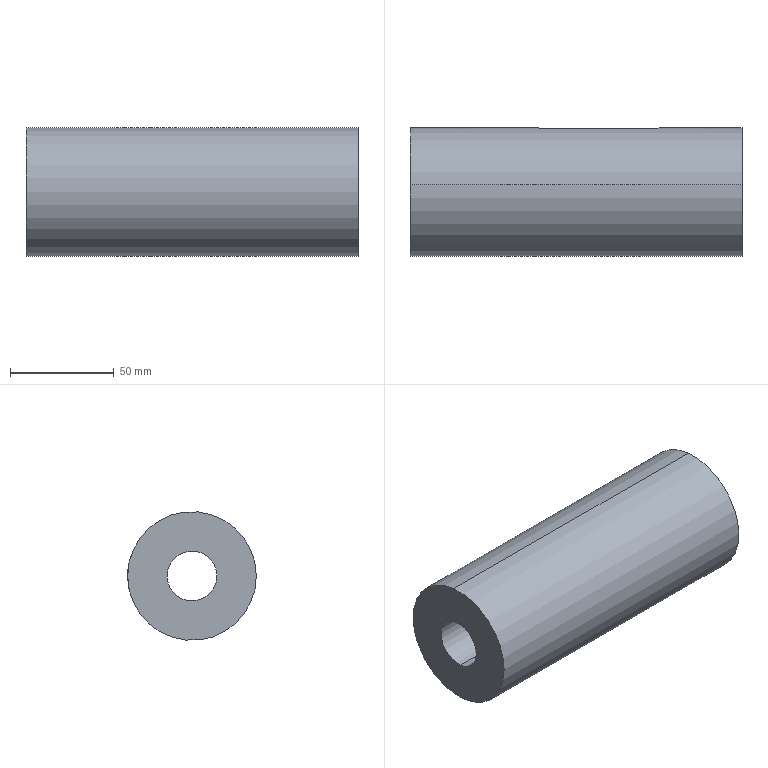Component | SolidWorks | Part4^LatheTailstock-1 | 1 solid | 17 faces | box 160 x 62 x 62 mm | volume 398970 mm3 | plane 9 | cylinder 8 | commonest cylinder face diameters 24 x4 30 x2 62 x2
STEP:
#1=CARTESIAN_POINT('',(-0.4506,5.972,-0.003713));
#2=VERTEX_POINT('',#1);
#3=CARTESIAN_POINT('',(-0.4506,5.839,-1.177));
#4=VERTEX_POINT('',#3);
#5=CARTESIAN_POINT('',(-0.4506,5.906,-0.5906));
#6=DIRECTION('',(1.,0.,0.));
#7=DIRECTION('',(0.,-0.112,-0.9937));
#8=AXIS2_PLACEMENT_3D('',#5,#6,#7);
#9=CIRCLE('',#8,0.5906);
#10=EDGE_CURVE('',#2,#4,#9,.T.);
#11=ORIENTED_EDGE('',*,*,#10,.F.);
#12=CARTESIAN_POINT('',(0.7305,5.972,-0.003713));
#13=VERTEX_POINT('',#12);
#14=CARTESIAN_POINT('',(-0.4506,5.972,-0.003713));
#15=DIRECTION('',(1.,0.,0.));
#16=VECTOR('',#15,39.37);
#17=LINE('',#14,#16);
#18=EDGE_CURVE('',#2,#13,#17,.T.);
#19=ORIENTED_EDGE('',*,*,#18,.T.);
#20=CARTESIAN_POINT('',(0.7305,5.839,-1.177));
#21=VERTEX_POINT('',#20);
#22=CARTESIAN_POINT('',(0.7305,5.906,-0.5906));
#23=DIRECTION('',(1.,0.,0.));
#24=DIRECTION('',(0.,-0.112,-0.9937));
#25=AXIS2_PLACEMENT_3D('',#22,#23,#24);
#26=CIRCLE('',#25,0.5906);
#27=EDGE_CURVE('',#13,#21,#26,.T.);
#28=ORIENTED_EDGE('',*,*,#27,.T.);
#29=CARTESIAN_POINT('',(-0.4506,5.839,-1.177));
#30=DIRECTION('',(1.,0.,0.));
#31=VECTOR('',#30,39.37);
#32=LINE('',#29,#31);
#33=EDGE_CURVE('',#4,#21,#32,.T.);
#34=ORIENTED_EDGE('',*,*,#33,.F.);
#35=EDGE_LOOP('',(#11,#19,#28,#34));
#36=FACE_OUTER_BOUND('',#35,.T.);
#37=CARTESIAN_POINT('',(-0.4506,5.906,-0.5906));
#38=DIRECTION('',(1.,0.,0.));
#39=DIRECTION('',(0.,-0.112,-0.9937));
#40=AXIS2_PLACEMENT_3D('',#37,#38,#39);
#41=CYLINDRICAL_SURFACE('',#40,0.5906);
#42=ADVANCED_FACE('',(#36),#41,.F.);
#43=CARTESIAN_POINT('',(0.7305,5.853,-1.06));
#44=VERTEX_POINT('',#43);
#45=CARTESIAN_POINT('',(0.7305,5.958,-0.1211));
#46=VERTEX_POINT('',#45);
#47=CARTESIAN_POINT('',(0.7305,5.906,-0.5906));
#48=DIRECTION('',(-1.,0.,0.));
#49=DIRECTION('',(0.,-0.112,-0.9937));
#50=AXIS2_PLACEMENT_3D('',#47,#48,#49);
#51=CIRCLE('',#50,0.4724);
#52=EDGE_CURVE('',#44,#46,#51,.T.);
#53=ORIENTED_EDGE('',*,*,#52,.T.);
#54=CARTESIAN_POINT('',(2.305,5.958,-0.1211));
#55=VERTEX_POINT('',#54);
#56=CARTESIAN_POINT('',(-3.207,5.958,-0.1211));
#57=DIRECTION('',(1.,0.,0.));
#58=VECTOR('',#57,39.37);
#59=LINE('',#56,#58);
#60=EDGE_CURVE('',#46,#55,#59,.T.);
#61=ORIENTED_EDGE('',*,*,#60,.T.);
#62=CARTESIAN_POINT('',(2.305,5.853,-1.06));
#63=VERTEX_POINT('',#62);
#64=CARTESIAN_POINT('',(2.305,5.906,-0.5906));
#65=DIRECTION('',(1.,0.,0.));
#66=DIRECTION('',(0.,-0.112,-0.9937));
#67=AXIS2_PLACEMENT_3D('',#64,#65,#66);
#68=CIRCLE('',#67,0.4724);
#69=EDGE_CURVE('',#55,#63,#68,.T.);
#70=ORIENTED_EDGE('',*,*,#69,.T.);
#71=CARTESIAN_POINT('',(-3.207,5.853,-1.06));
#72=DIRECTION('',(1.,0.,0.));
#73=VECTOR('',#72,39.37);
#74=LINE('',#71,#73);
#75=EDGE_CURVE('',#44,#63,#74,.T.);
#76=ORIENTED_EDGE('',*,*,#75,.F.);
#77=EDGE_LOOP('',(#53,#61,#70,#76));
#78=FACE_OUTER_BOUND('',#77,.T.);
#79=CARTESIAN_POINT('',(-3.207,5.906,-0.5906));
#80=DIRECTION('',(1.,0.,0.));
#81=DIRECTION('',(0.,-0.112,-0.9937));
#82=AXIS2_PLACEMENT_3D('',#79,#80,#81);
#83=CYLINDRICAL_SURFACE('',#82,0.4724);
#84=ADVANCED_FACE('',(#78),#83,.F.);
#85=CARTESIAN_POINT('',(-3.994,5.853,-1.06));
#86=VERTEX_POINT('',#85);
#87=CARTESIAN_POINT('',(-3.994,5.958,-0.1211));
#88=VERTEX_POINT('',#87);
#89=CARTESIAN_POINT('',(-3.994,5.906,-0.5906));
#90=DIRECTION('',(-1.,0.,0.));
#91=DIRECTION('',(0.,0.112,0.9937));
#92=AXIS2_PLACEMENT_3D('',#89,#90,#91);
#93=CIRCLE('',#92,0.4724);
#94=EDGE_CURVE('',#86,#88,#93,.T.);
#95=ORIENTED_EDGE('',*,*,#94,.T.);
#96=CARTESIAN_POINT('',(-0.4506,5.958,-0.1211));
#97=VERTEX_POINT('',#96);
#98=CARTESIAN_POINT('',(-3.207,5.958,-0.1211));
#99=DIRECTION('',(1.,0.,0.));
#100=VECTOR('',#99,39.37);
#101=LINE('',#98,#100);
#102=EDGE_CURVE('',#88,#97,#101,.T.);
#103=ORIENTED_EDGE('',*,*,#102,.T.);
#104=CARTESIAN_POINT('',(-0.4506,5.853,-1.06));
#105=VERTEX_POINT('',#104);
#106=CARTESIAN_POINT('',(-0.4506,5.906,-0.5906));
#107=DIRECTION('',(-1.,0.,0.));
#108=DIRECTION('',(0.,-0.112,-0.9937));
#109=AXIS2_PLACEMENT_3D('',#106,#107,#108);
#110=CIRCLE('',#109,0.4724);
#111=EDGE_CURVE('',#105,#97,#110,.T.);
#112=ORIENTED_EDGE('',*,*,#111,.F.);
#113=CARTESIAN_POINT('',(-3.207,5.853,-1.06));
#114=DIRECTION('',(1.,0.,0.));
#115=VECTOR('',#114,39.37);
#116=LINE('',#113,#115);
#117=EDGE_CURVE('',#86,#105,#116,.T.);
#118=ORIENTED_EDGE('',*,*,#117,.F.);
#119=EDGE_LOOP('',(#95,#103,#112,#118));
#120=FACE_OUTER_BOUND('',#119,.T.);
#121=CARTESIAN_POINT('',(-3.207,5.906,-0.5906));
#122=DIRECTION('',(1.,0.,0.));
#123=DIRECTION('',(0.,-0.112,-0.9937));
#124=AXIS2_PLACEMENT_3D('',#121,#122,#123);
#125=CYLINDRICAL_SURFACE('',#124,0.4724);
#126=ADVANCED_FACE('',(#120),#125,.F.);
#127=CARTESIAN_POINT('',(-1.553,7.096,-0.3206));
#128=VERTEX_POINT('',#127);
#129=CARTESIAN_POINT('',(0.7305,7.096,-0.3206));
#130=VERTEX_POINT('',#129);
#131=CARTESIAN_POINT('',(-3.207,7.096,-0.3206));
#132=DIRECTION('',(1.,0.,0.));
#133=VECTOR('',#132,39.37);
#134=LINE('',#131,#133);
#135=EDGE_CURVE('',#128,#130,#134,.T.);
#136=ORIENTED_EDGE('',*,*,#135,.F.);
#137=CARTESIAN_POINT('',(-1.553,7.112,-0.7755));
#138=VERTEX_POINT('',#137);
#139=CARTESIAN_POINT('',(-1.553,5.906,-0.5906));
#140=DIRECTION('',(-1.,0.,0.));
#141=DIRECTION('',(0.,-0.112,-0.9937));
#142=AXIS2_PLACEMENT_3D('',#139,#140,#141);
#143=CIRCLE('',#142,1.22);
#144=EDGE_CURVE('',#128,#138,#143,.T.);
#145=ORIENTED_EDGE('',*,*,#144,.T.);
#146=CARTESIAN_POINT('',(0.7305,7.112,-0.7755));
#147=VERTEX_POINT('',#146);
#148=CARTESIAN_POINT('',(-3.207,7.112,-0.7755));
#149=DIRECTION('',(-1.,0.,0.));
#150=VECTOR('',#149,39.37);
#151=LINE('',#148,#150);
#152=EDGE_CURVE('',#147,#138,#151,.T.);
#153=ORIENTED_EDGE('',*,*,#152,.F.);
#154=CARTESIAN_POINT('',(0.7305,5.906,-0.5906));
#155=DIRECTION('',(-1.,0.,0.));
#156=DIRECTION('',(0.,-0.112,-0.9937));
#157=AXIS2_PLACEMENT_3D('',#154,#155,#156);
#158=CIRCLE('',#157,1.22);
#159=EDGE_CURVE('',#130,#147,#158,.T.);
#160=ORIENTED_EDGE('',*,*,#159,.F.);
#161=EDGE_LOOP('',(#136,#145,#153,#160));
#162=FACE_BOUND('',#161,.T.);
#163=CARTESIAN_POINT('',(-3.994,6.042,0.6222));
#164=VERTEX_POINT('',#163);
#165=CARTESIAN_POINT('',(-3.994,5.769,-1.803));
#166=VERTEX_POINT('',#165);
#167=CARTESIAN_POINT('',(-3.994,5.906,-0.5906));
#168=DIRECTION('',(-1.,0.,0.));
#169=DIRECTION('',(0.,0.112,0.9937));
#170=AXIS2_PLACEMENT_3D('',#167,#168,#169);
#171=CIRCLE('',#170,1.22);
#172=EDGE_CURVE('',#164,#166,#171,.T.);
#173=ORIENTED_EDGE('',*,*,#172,.F.);
#174=CARTESIAN_POINT('',(2.305,6.042,0.6222));
#175=VERTEX_POINT('',#174);
#176=CARTESIAN_POINT('',(-3.207,6.042,0.6222));
#177=DIRECTION('',(1.,0.,0.));
#178=VECTOR('',#177,39.37);
#179=LINE('',#176,#178);
#180=EDGE_CURVE('',#164,#175,#179,.T.);
#181=ORIENTED_EDGE('',*,*,#180,.T.);
#182=CARTESIAN_POINT('',(2.305,5.769,-1.803));
#183=VERTEX_POINT('',#182);
#184=CARTESIAN_POINT('',(2.305,5.906,-0.5906));
#185=DIRECTION('',(1.,0.,0.));
#186=DIRECTION('',(0.,-0.112,-0.9937));
#187=AXIS2_PLACEMENT_3D('',#184,#185,#186);
#188=CIRCLE('',#187,1.22);
#189=EDGE_CURVE('',#183,#175,#188,.T.);
#190=ORIENTED_EDGE('',*,*,#189,.F.);
#191=CARTESIAN_POINT('',(-3.207,5.769,-1.803));
#192=DIRECTION('',(1.,0.,0.));
#193=VECTOR('',#192,39.37);
#194=LINE('',#191,#193);
#195=EDGE_CURVE('',#166,#183,#194,.T.);
#196=ORIENTED_EDGE('',*,*,#195,.F.);
#197=EDGE_LOOP('',(#173,#181,#190,#196));
#198=FACE_OUTER_BOUND('',#197,.T.);
#199=CARTESIAN_POINT('',(-3.207,5.906,-0.5906));
#200=DIRECTION('',(1.,0.,0.));
#201=DIRECTION('',(0.,-0.112,-0.9937));
#202=AXIS2_PLACEMENT_3D('',#199,#200,#201);
#203=CYLINDRICAL_SURFACE('',#202,1.22);
#204=ADVANCED_FACE('',(#162,#198),#203,.T.);
#205=ORIENTED_EDGE('',*,*,#180,.F.);
#206=CARTESIAN_POINT('',(-3.994,5.906,-0.5906));
#207=DIRECTION('',(-1.,0.,0.));
#208=DIRECTION('',(0.,0.112,0.9937));
#209=AXIS2_PLACEMENT_3D('',#206,#207,#208);
#210=CIRCLE('',#209,1.22);
#211=EDGE_CURVE('',#166,#164,#210,.T.);
#212=ORIENTED_EDGE('',*,*,#211,.F.);
#213=ORIENTED_EDGE('',*,*,#195,.T.);
#214=CARTESIAN_POINT('',(2.305,5.906,-0.5906));
#215=DIRECTION('',(1.,0.,0.));
#216=DIRECTION('',(0.,-0.112,-0.9937));
#217=AXIS2_PLACEMENT_3D('',#214,#215,#216);
#218=CIRCLE('',#217,1.22);
#219=EDGE_CURVE('',#175,#183,#218,.T.);
#220=ORIENTED_EDGE('',*,*,#219,.F.);
#221=EDGE_LOOP('',(#205,#212,#213,#220));
#222=FACE_OUTER_BOUND('',#221,.T.);
#223=CARTESIAN_POINT('',(-3.207,5.906,-0.5906));
#224=DIRECTION('',(1.,0.,0.));
#225=DIRECTION('',(0.,-0.112,-0.9937));
#226=AXIS2_PLACEMENT_3D('',#223,#224,#225);
#227=CYLINDRICAL_SURFACE('',#226,1.22);
#228=ADVANCED_FACE('',(#222),#227,.T.);
#229=ORIENTED_EDGE('',*,*,#102,.F.);
#230=CARTESIAN_POINT('',(-3.994,5.906,-0.5906));
#231=DIRECTION('',(-1.,0.,0.));
#232=DIRECTION('',(0.,0.112,0.9937));
#233=AXIS2_PLACEMENT_3D('',#230,#231,#232);
#234=CIRCLE('',#233,0.4724);
#235=EDGE_CURVE('',#88,#86,#234,.T.);
#236=ORIENTED_EDGE('',*,*,#235,.T.);
#237=ORIENTED_EDGE('',*,*,#117,.T.);
#238=CARTESIAN_POINT('',(-0.4506,5.906,-0.5906));
#239=DIRECTION('',(-1.,0.,0.));
#240=DIRECTION('',(0.,-0.112,-0.9937));
#241=AXIS2_PLACEMENT_3D('',#238,#239,#240);
#242=CIRCLE('',#241,0.4724);
#243=EDGE_CURVE('',#97,#105,#242,.T.);
#244=ORIENTED_EDGE('',*,*,#243,.F.);
#245=EDGE_LOOP('',(#229,#236,#237,#244));
#246=FACE_OUTER_BOUND('',#245,.T.);
#247=CARTESIAN_POINT('',(-3.207,5.906,-0.5906));
#248=DIRECTION('',(1.,0.,0.));
#249=DIRECTION('',(0.,-0.112,-0.9937));
#250=AXIS2_PLACEMENT_3D('',#247,#248,#249);
#251=CYLINDRICAL_SURFACE('',#250,0.4724);
#252=ADVANCED_FACE('',(#246),#251,.F.);
#253=ORIENTED_EDGE('',*,*,#60,.F.);
#254=CARTESIAN_POINT('',(0.7305,5.906,-0.5906));
#255=DIRECTION('',(-1.,0.,0.));
#256=DIRECTION('',(0.,-0.112,-0.9937));
#257=AXIS2_PLACEMENT_3D('',#254,#255,#256);
#258=CIRCLE('',#257,0.4724);
#259=EDGE_CURVE('',#46,#44,#258,.T.);
#260=ORIENTED_EDGE('',*,*,#259,.T.);
#261=ORIENTED_EDGE('',*,*,#75,.T.);
#262=CARTESIAN_POINT('',(2.305,5.906,-0.5906));
#263=DIRECTION('',(1.,0.,0.));
#264=DIRECTION('',(0.,-0.112,-0.9937));
#265=AXIS2_PLACEMENT_3D('',#262,#263,#264);
#266=CIRCLE('',#265,0.4724);
#267=EDGE_CURVE('',#63,#55,#266,.T.);
#268=ORIENTED_EDGE('',*,*,#267,.T.);
#269=EDGE_LOOP('',(#253,#260,#261,#268));
#270=FACE_OUTER_BOUND('',#269,.T.);
#271=CARTESIAN_POINT('',(-3.207,5.906,-0.5906));
#272=DIRECTION('',(1.,0.,0.));
#273=DIRECTION('',(0.,-0.112,-0.9937));
#274=AXIS2_PLACEMENT_3D('',#271,#272,#273);
#275=CYLINDRICAL_SURFACE('',#274,0.4724);
#276=ADVANCED_FACE('',(#270),#275,.F.);
#277=CARTESIAN_POINT('',(-0.4506,5.906,-0.5906));
#278=DIRECTION('',(1.,0.,0.));
#279=DIRECTION('',(0.,-0.112,-0.9937));
#280=AXIS2_PLACEMENT_3D('',#277,#278,#279);
#281=CIRCLE('',#280,0.5906);
#282=EDGE_CURVE('',#4,#2,#281,.T.);
#283=ORIENTED_EDGE('',*,*,#282,.T.);
#284=ORIENTED_EDGE('',*,*,#10,.T.);
#285=EDGE_LOOP('',(#283,#284));
#286=FACE_OUTER_BOUND('',#285,.T.);
#287=ORIENTED_EDGE('',*,*,#111,.T.);
#288=ORIENTED_EDGE('',*,*,#243,.T.);
#289=EDGE_LOOP('',(#287,#288));
#290=FACE_BOUND('',#289,.T.);
#291=CARTESIAN_POINT('',(-0.4506,5.906,-0.5906));
#292=DIRECTION('',(1.,0.,0.));
#293=DIRECTION('',(0.,-0.112,-0.9937));
#294=AXIS2_PLACEMENT_3D('',#291,#292,#293);
#295=PLANE('',#294);
#296=ADVANCED_FACE('',(#286,#290),#295,.T.);
#297=CARTESIAN_POINT('',(0.7305,5.906,-0.5906));
#298=DIRECTION('',(1.,0.,0.));
#299=DIRECTION('',(0.,-0.112,-0.9937));
#300=AXIS2_PLACEMENT_3D('',#297,#298,#299);
#301=CIRCLE('',#300,0.5906);
#302=EDGE_CURVE('',#21,#13,#301,.T.);
#303=ORIENTED_EDGE('',*,*,#302,.F.);
#304=ORIENTED_EDGE('',*,*,#27,.F.);
#305=EDGE_LOOP('',(#303,#304));
#306=FACE_OUTER_BOUND('',#305,.T.);
#307=ORIENTED_EDGE('',*,*,#52,.F.);
#308=ORIENTED_EDGE('',*,*,#259,.F.);
#309=EDGE_LOOP('',(#307,#308));
#310=FACE_BOUND('',#309,.T.);
#311=CARTESIAN_POINT('',(0.7305,5.906,-0.5906));
#312=DIRECTION('',(1.,0.,0.));
#313=DIRECTION('',(0.,-0.112,-0.9937));
#314=AXIS2_PLACEMENT_3D('',#311,#312,#313);
#315=PLANE('',#314);
#316=ADVANCED_FACE('',(#306,#310),#315,.F.);
#317=ORIENTED_EDGE('',*,*,#18,.F.);
#318=ORIENTED_EDGE('',*,*,#282,.F.);
#319=ORIENTED_EDGE('',*,*,#33,.T.);
#320=ORIENTED_EDGE('',*,*,#302,.T.);
#321=EDGE_LOOP('',(#317,#318,#319,#320));
#322=FACE_OUTER_BOUND('',#321,.T.);
#323=CARTESIAN_POINT('',(-0.4506,5.906,-0.5906));
#324=DIRECTION('',(1.,0.,0.));
#325=DIRECTION('',(0.,-0.112,-0.9937));
#326=AXIS2_PLACEMENT_3D('',#323,#324,#325);
#327=CYLINDRICAL_SURFACE('',#326,0.5906);
#328=ADVANCED_FACE('',(#322),#327,.F.);
#329=ORIENTED_EDGE('',*,*,#152,.T.);
#330=CARTESIAN_POINT('',(-1.553,6.888,-0.7835));
#331=VERTEX_POINT('',#330);
#332=CARTESIAN_POINT('',(-1.553,7.11,-0.7756));
#333=DIRECTION('',(0.,0.9994,0.03535));
#334=VECTOR('',#333,39.37);
#335=LINE('',#332,#334);
#336=EDGE_CURVE('',#331,#138,#335,.T.);
#337=ORIENTED_EDGE('',*,*,#336,.F.);
#338=CARTESIAN_POINT('',(0.7305,6.888,-0.7835));
#339=VERTEX_POINT('',#338);
#340=CARTESIAN_POINT('',(-1.553,6.888,-0.7835));
#341=DIRECTION('',(1.,0.,0.));
#342=VECTOR('',#341,39.37);
#343=LINE('',#340,#342);
#344=EDGE_CURVE('',#331,#339,#343,.T.);
#345=ORIENTED_EDGE('',*,*,#344,.T.);
#346=CARTESIAN_POINT('',(0.7305,7.366,-0.7665));
#347=DIRECTION('',(0.,0.9994,0.03535));
#348=VECTOR('',#347,39.37);
#349=LINE('',#346,#348);
#350=EDGE_CURVE('',#339,#147,#349,.T.);
#351=ORIENTED_EDGE('',*,*,#350,.T.);
#352=EDGE_LOOP('',(#329,#337,#345,#351));
#353=FACE_OUTER_BOUND('',#352,.T.);
#354=CARTESIAN_POINT('',(-1.553,7.366,-0.7665));
#355=DIRECTION('',(0.,0.03535,-0.9994));
#356=DIRECTION('',(0.,0.9994,0.03535));
#357=AXIS2_PLACEMENT_3D('',#354,#355,#356);
#358=PLANE('',#357);
#359=ADVANCED_FACE('',(#353),#358,.F.);
#360=CARTESIAN_POINT('',(0.7305,6.872,-0.3286));
#361=VERTEX_POINT('',#360);
#362=CARTESIAN_POINT('',(0.7305,6.872,-0.3286));
#363=DIRECTION('',(0.,0.03535,-0.9994));
#364=VECTOR('',#363,39.37);
#365=LINE('',#362,#364);
#366=EDGE_CURVE('',#361,#339,#365,.T.);
#367=ORIENTED_EDGE('',*,*,#366,.T.);
#368=ORIENTED_EDGE('',*,*,#344,.F.);
#369=CARTESIAN_POINT('',(-1.553,6.872,-0.3286));
#370=VERTEX_POINT('',#369);
#371=CARTESIAN_POINT('',(-1.553,6.872,-0.3286));
#372=DIRECTION('',(0.,0.03535,-0.9994));
#373=VECTOR('',#372,39.37);
#374=LINE('',#371,#373);
#375=EDGE_CURVE('',#370,#331,#374,.T.);
#376=ORIENTED_EDGE('',*,*,#375,.F.);
#377=CARTESIAN_POINT('',(-1.553,6.872,-0.3286));
#378=DIRECTION('',(1.,0.,0.));
#379=VECTOR('',#378,39.37);
#380=LINE('',#377,#379);
#381=EDGE_CURVE('',#370,#361,#380,.T.);
#382=ORIENTED_EDGE('',*,*,#381,.T.);
#383=EDGE_LOOP('',(#367,#368,#376,#382));
#384=FACE_OUTER_BOUND('',#383,.T.);
#385=CARTESIAN_POINT('',(-1.553,6.872,-0.3286));
#386=DIRECTION('',(0.,-0.9994,-0.03535));
#387=DIRECTION('',(0.,0.03535,-0.9994));
#388=AXIS2_PLACEMENT_3D('',#385,#386,#387);
#389=PLANE('',#388);
#390=ADVANCED_FACE('',(#384),#389,.F.);
#391=ORIENTED_EDGE('',*,*,#135,.T.);
#392=CARTESIAN_POINT('',(0.7305,7.094,-0.3207));
#393=DIRECTION('',(0.,-0.9994,-0.03535));
#394=VECTOR('',#393,39.37);
#395=LINE('',#392,#394);
#396=EDGE_CURVE('',#130,#361,#395,.T.);
#397=ORIENTED_EDGE('',*,*,#396,.T.);
#398=ORIENTED_EDGE('',*,*,#381,.F.);
#399=CARTESIAN_POINT('',(-1.553,7.35,-0.3116));
#400=DIRECTION('',(0.,-0.9994,-0.03535));
#401=VECTOR('',#400,39.37);
#402=LINE('',#399,#401);
#403=EDGE_CURVE('',#128,#370,#402,.T.);
#404=ORIENTED_EDGE('',*,*,#403,.F.);
#405=EDGE_LOOP('',(#391,#397,#398,#404));
#406=FACE_OUTER_BOUND('',#405,.T.);
#407=CARTESIAN_POINT('',(-1.553,7.094,-0.3207));
#408=DIRECTION('',(0.,-0.03535,0.9994));
#409=DIRECTION('',(0.,-0.9994,-0.03535));
#410=AXIS2_PLACEMENT_3D('',#407,#408,#409);
#411=PLANE('',#410);
#412=ADVANCED_FACE('',(#406),#411,.F.);
#413=ORIENTED_EDGE('',*,*,#403,.T.);
#414=ORIENTED_EDGE('',*,*,#375,.T.);
#415=ORIENTED_EDGE('',*,*,#336,.T.);
#416=ORIENTED_EDGE('',*,*,#144,.F.);
#417=EDGE_LOOP('',(#413,#414,#415,#416));
#418=FACE_OUTER_BOUND('',#417,.T.);
#419=CARTESIAN_POINT('',(-1.553,-0.5167,0.7908));
#420=DIRECTION('',(1.,0.,0.));
#421=DIRECTION('',(0.,-0.112,-0.9937));
#422=AXIS2_PLACEMENT_3D('',#419,#420,#421);
#423=PLANE('',#422);
#424=ADVANCED_FACE('',(#418),#423,.T.);
#425=ORIENTED_EDGE('',*,*,#159,.T.);
#426=ORIENTED_EDGE('',*,*,#350,.F.);
#427=ORIENTED_EDGE('',*,*,#366,.F.);
#428=ORIENTED_EDGE('',*,*,#396,.F.);
#429=EDGE_LOOP('',(#425,#426,#427,#428));
#430=FACE_OUTER_BOUND('',#429,.T.);
#431=CARTESIAN_POINT('',(0.7305,-0.5167,0.7908));
#432=DIRECTION('',(1.,0.,0.));
#433=DIRECTION('',(0.,-0.112,-0.9937));
#434=AXIS2_PLACEMENT_3D('',#431,#432,#433);
#435=PLANE('',#434);
#436=ADVANCED_FACE('',(#430),#435,.F.);
#437=ORIENTED_EDGE('',*,*,#211,.T.);
#438=ORIENTED_EDGE('',*,*,#172,.T.);
#439=EDGE_LOOP('',(#437,#438));
#440=FACE_OUTER_BOUND('',#439,.T.);
#441=ORIENTED_EDGE('',*,*,#94,.F.);
#442=ORIENTED_EDGE('',*,*,#235,.F.);
#443=EDGE_LOOP('',(#441,#442));
#444=FACE_BOUND('',#443,.T.);
#445=CARTESIAN_POINT('',(-3.994,5.906,-0.5906));
#446=DIRECTION('',(-1.,0.,0.));
#447=DIRECTION('',(0.,0.112,0.9937));
#448=AXIS2_PLACEMENT_3D('',#445,#446,#447);
#449=PLANE('',#448);
#450=ADVANCED_FACE('',(#440,#444),#449,.T.);
#451=ORIENTED_EDGE('',*,*,#189,.T.);
#452=ORIENTED_EDGE('',*,*,#219,.T.);
#453=EDGE_LOOP('',(#451,#452));
#454=FACE_OUTER_BOUND('',#453,.T.);
#455=ORIENTED_EDGE('',*,*,#267,.F.);
#456=ORIENTED_EDGE('',*,*,#69,.F.);
#457=EDGE_LOOP('',(#455,#456));
#458=FACE_BOUND('',#457,.T.);
#459=CARTESIAN_POINT('',(2.305,5.906,-0.5906));
#460=DIRECTION('',(1.,0.,0.));
#461=DIRECTION('',(0.,-0.112,-0.9937));
#462=AXIS2_PLACEMENT_3D('',#459,#460,#461);
#463=PLANE('',#462);
#464=ADVANCED_FACE('',(#454,#458),#463,.T.);
#465=CLOSED_SHELL('',(#42,#84,#126,#204,#228,#252,#276,#296,#316,#328,#359,#390,#412,#424,#436,#450,#464));
#466=MANIFOLD_SOLID_BREP('',#465);
#467=CARTESIAN_POINT('',(0.,0.,0.));
#468=DIRECTION('',(0.,0.,1.));
#469=DIRECTION('',(1.,0.,0.));
#470=AXIS2_PLACEMENT_3D('',#467,#468,#469);
#471=(LENGTH_UNIT()NAMED_UNIT(*)SI_UNIT($,.METRE.));
#472=LENGTH_MEASURE_WITH_UNIT(LENGTH_MEASURE(0.0254),#471);
#473=DIMENSIONAL_EXPONENTS(1.,0.,0.,0.,0.,0.,0.);
#474=(CONVERSION_BASED_UNIT('',#472)LENGTH_UNIT()NAMED_UNIT(#473));
#475=UNCERTAINTY_MEASURE_WITH_UNIT(LENGTH_MEASURE(0.00001),#474,'','');
#476=(NAMED_UNIT(*)PLANE_ANGLE_UNIT()SI_UNIT($,.RADIAN.));
#477=(NAMED_UNIT(*)SI_UNIT($,.STERADIAN.)SOLID_ANGLE_UNIT());
#478=(GEOMETRIC_REPRESENTATION_CONTEXT(3)GLOBAL_UNCERTAINTY_ASSIGNED_CONTEXT((#475))GLOBAL_UNIT_ASSIGNED_CONTEXT((#474,#476,#477))REPRESENTATION_CONTEXT('',''));
#479=ADVANCED_BREP_SHAPE_REPRESENTATION('',(#466,#470),#478);
#480=COLOUR_RGB('',0.7922,0.8196,0.9333);
#481=FILL_AREA_STYLE_COLOUR('',#480);
#482=FILL_AREA_STYLE('',(#481));
#483=SURFACE_STYLE_FILL_AREA(#482);
#484=SURFACE_SIDE_STYLE('',(#483));
#485=SURFACE_STYLE_USAGE(.BOTH.,#484);
#486=PRESENTATION_STYLE_ASSIGNMENT((#485));
#487=STYLED_ITEM('',(#486),#466);
#488=PRESENTATION_LAYER_ASSIGNMENT('','',(#487));
#489=(LENGTH_UNIT()NAMED_UNIT(*)SI_UNIT($,.METRE.));
#490=LENGTH_MEASURE_WITH_UNIT(LENGTH_MEASURE(0.0254),#489);
#491=DIMENSIONAL_EXPONENTS(1.,0.,0.,0.,0.,0.,0.);
#492=(CONVERSION_BASED_UNIT('',#490)LENGTH_UNIT()NAMED_UNIT(#491));
#493=UNCERTAINTY_MEASURE_WITH_UNIT(LENGTH_MEASURE(0.00001),#492,'','');
#494=(NAMED_UNIT(*)PLANE_ANGLE_UNIT()SI_UNIT($,.RADIAN.));
#495=(NAMED_UNIT(*)SI_UNIT($,.STERADIAN.)SOLID_ANGLE_UNIT());
#496=(GEOMETRIC_REPRESENTATION_CONTEXT(3)GLOBAL_UNCERTAINTY_ASSIGNED_CONTEXT((#493))GLOBAL_UNIT_ASSIGNED_CONTEXT((#492,#494,#495))REPRESENTATION_CONTEXT('',''));
#497=MECHANICAL_DESIGN_GEOMETRIC_PRESENTATION_REPRESENTATION('',(#487),#496);